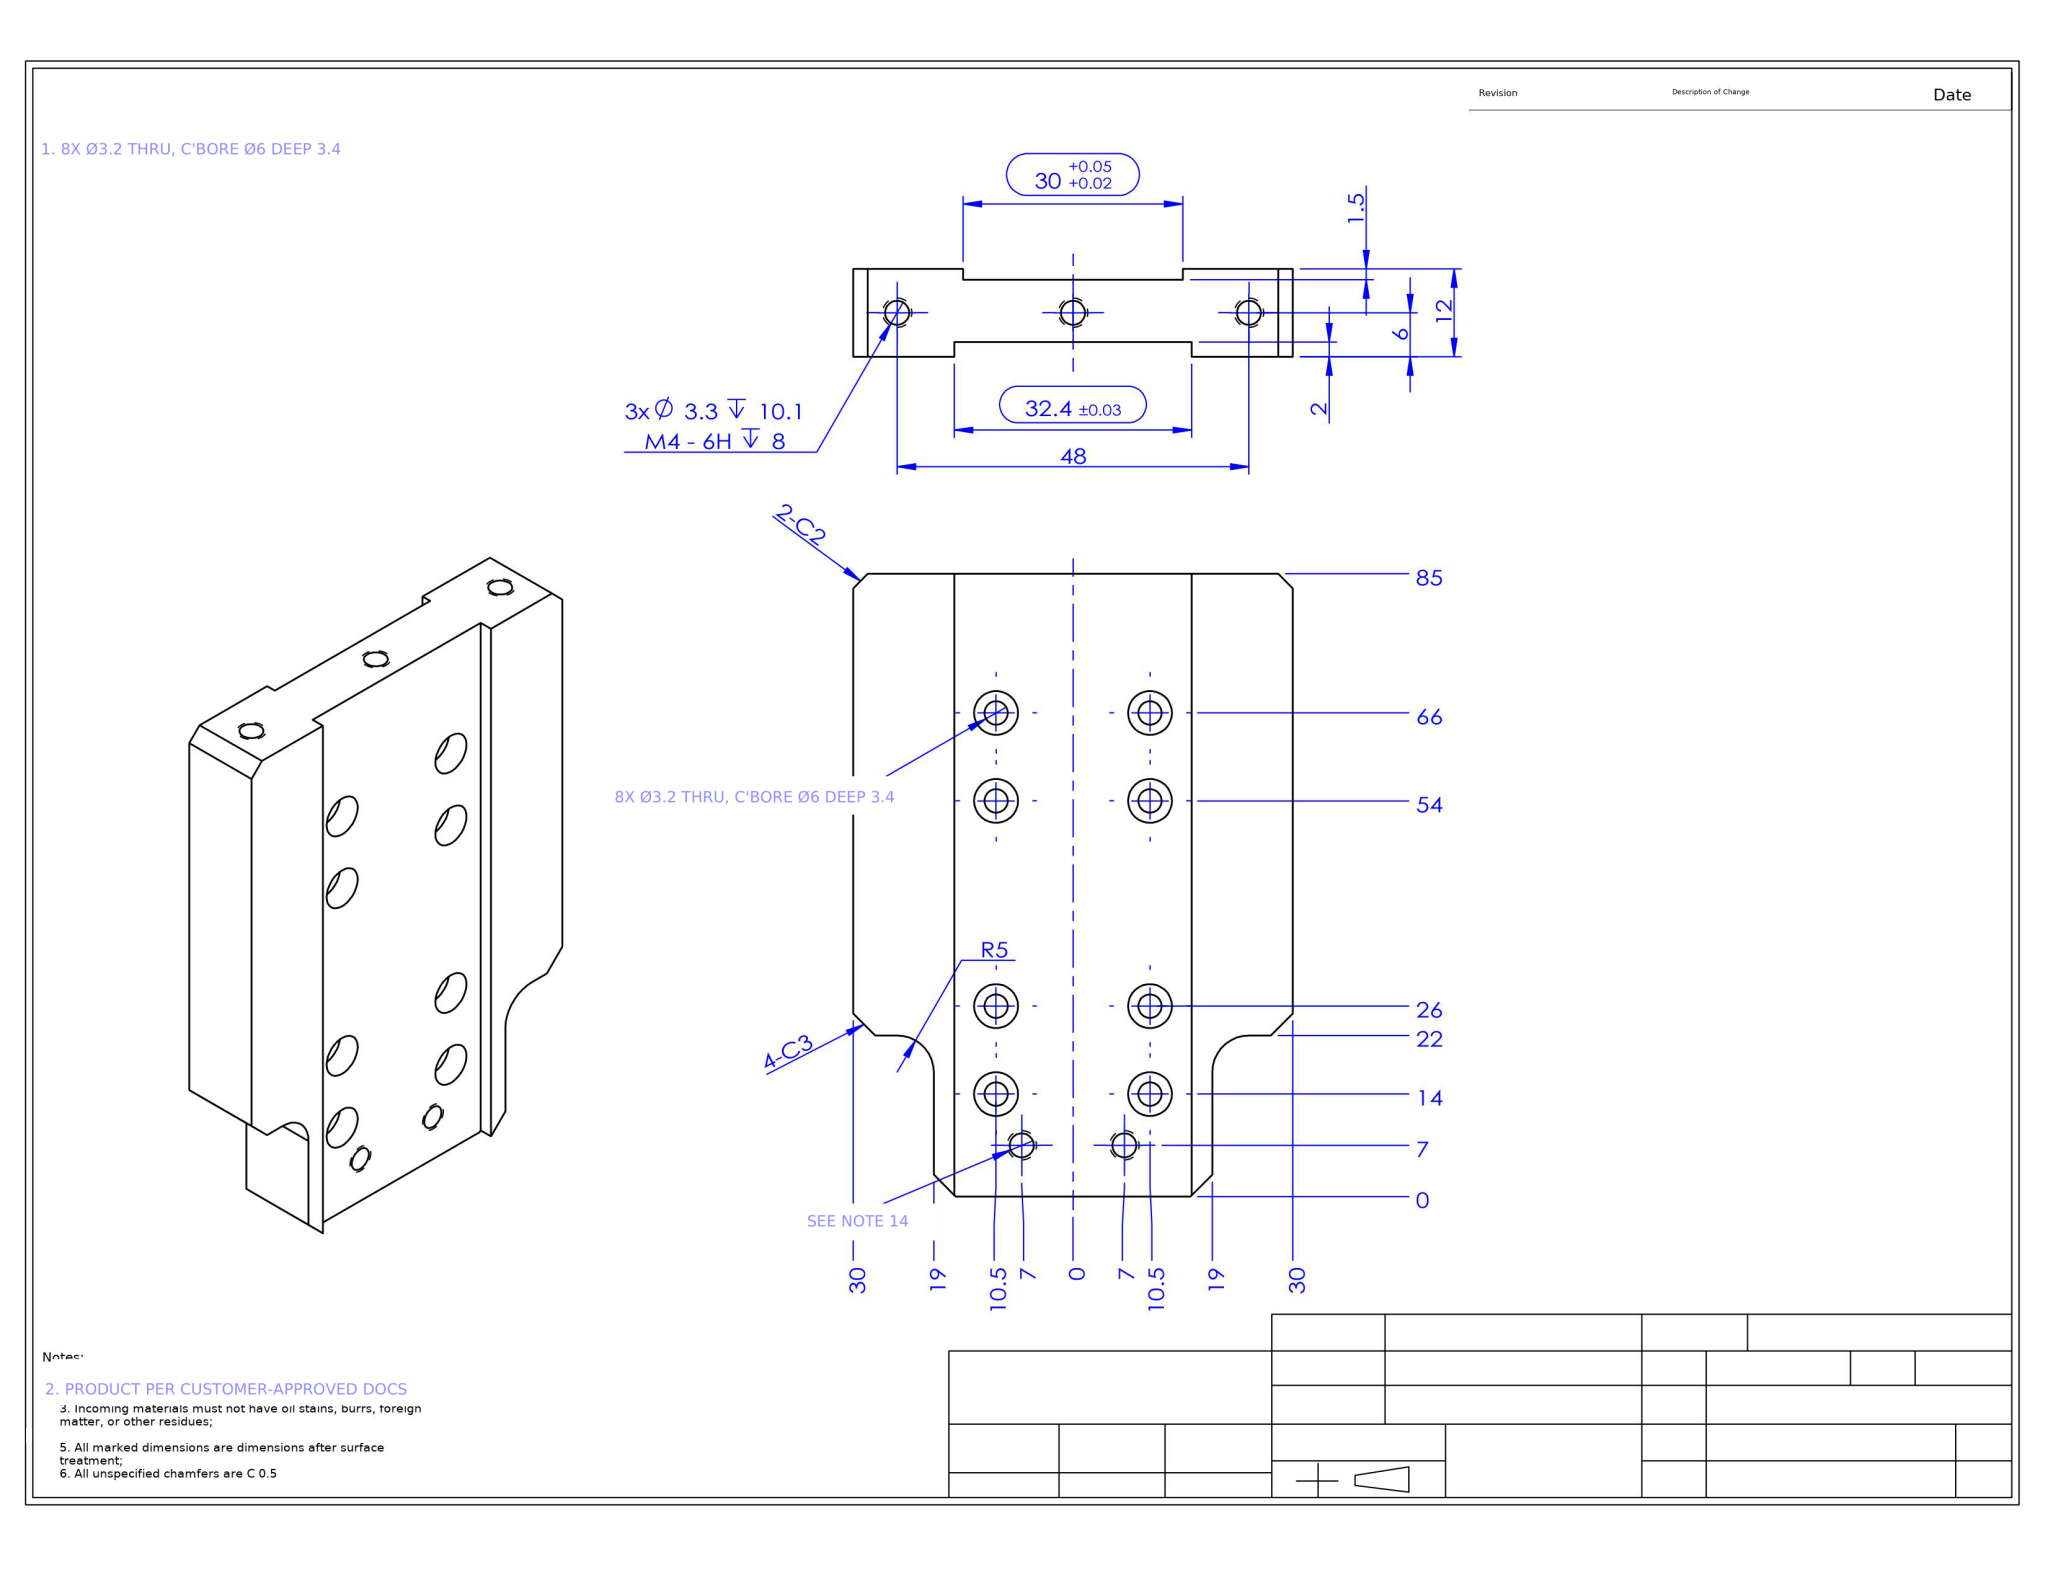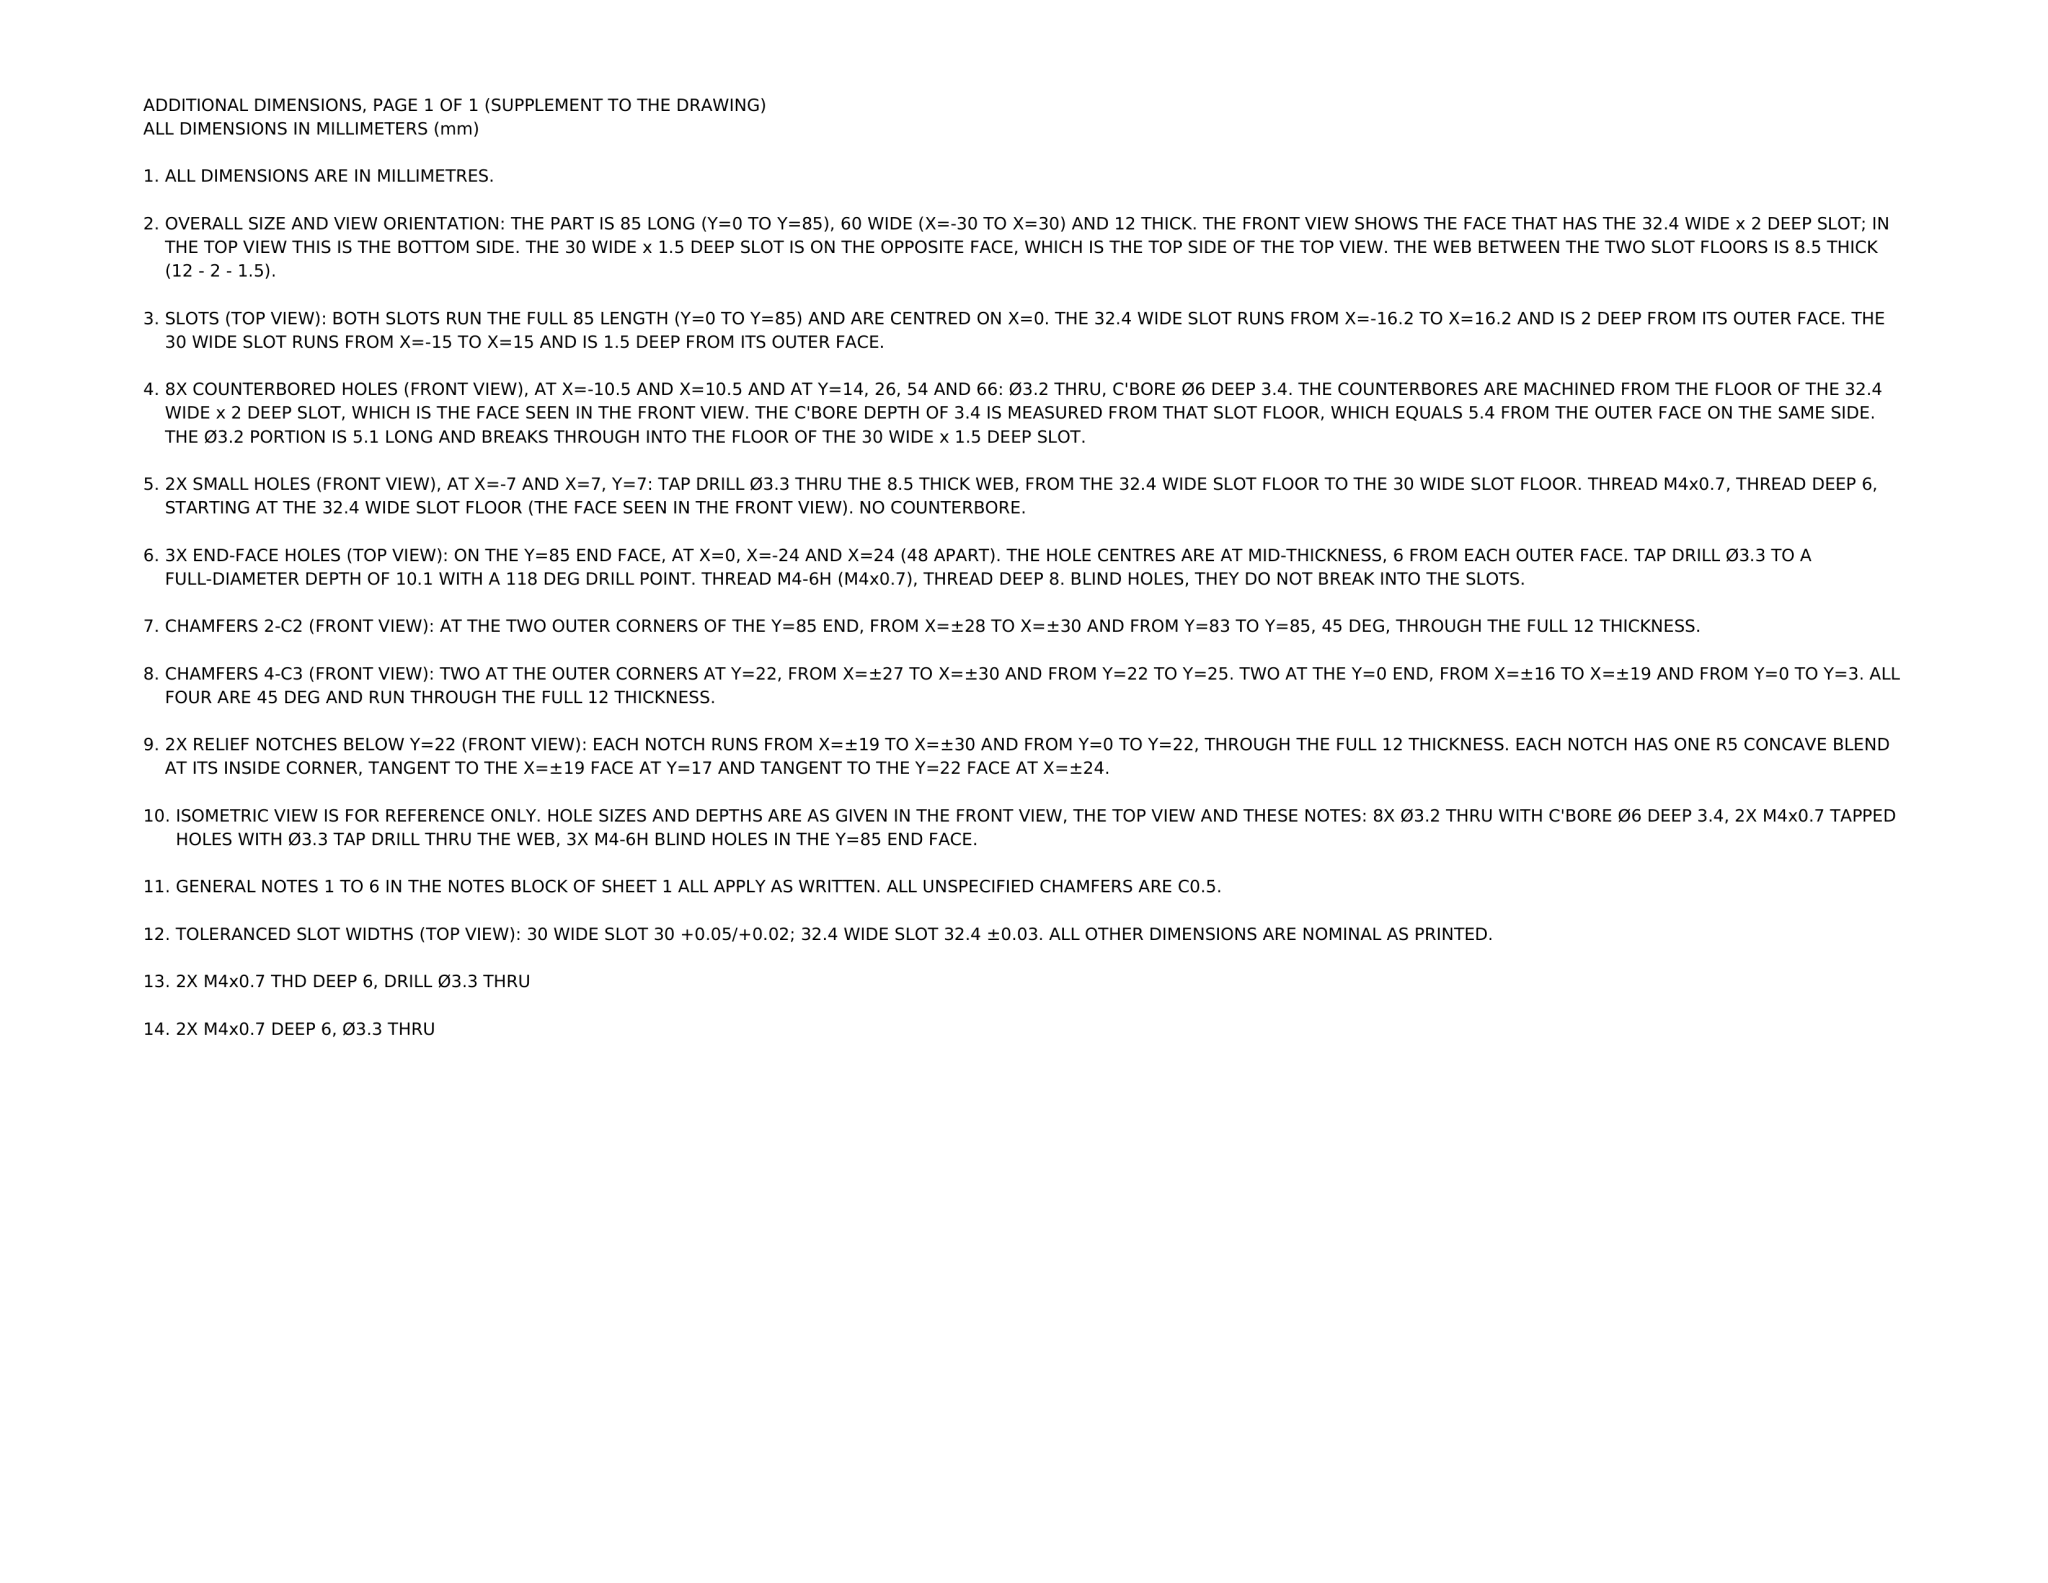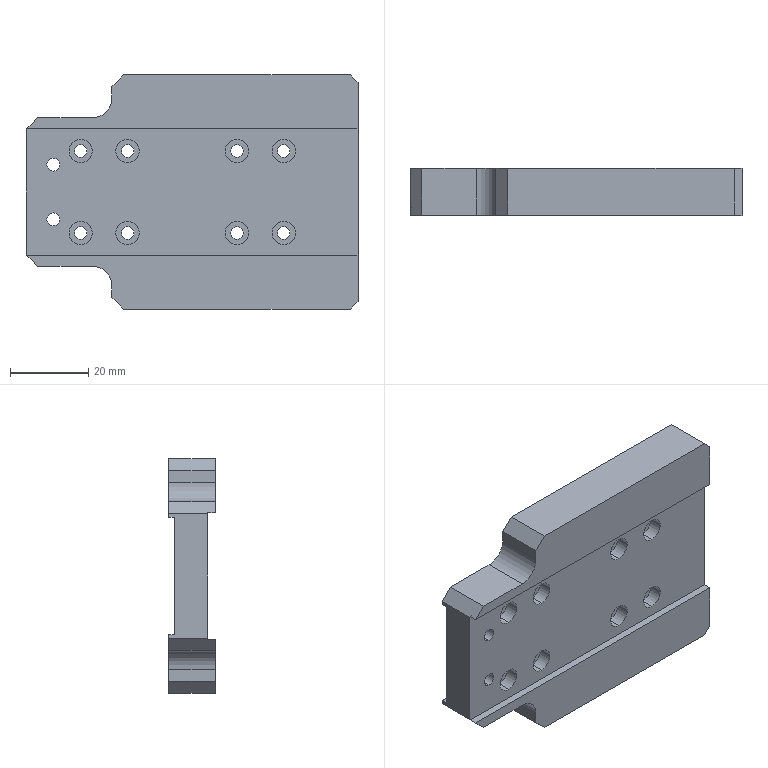Part | NX | mm | 1 solid | 82 faces | box 85 x 12 x 60 mm | volume 44414 mm3 | cylinder 44 | plane 32 | cone 6 | commonest cylinder face diameters 3.2 x16 6 x16 3.3 x10 10 x2